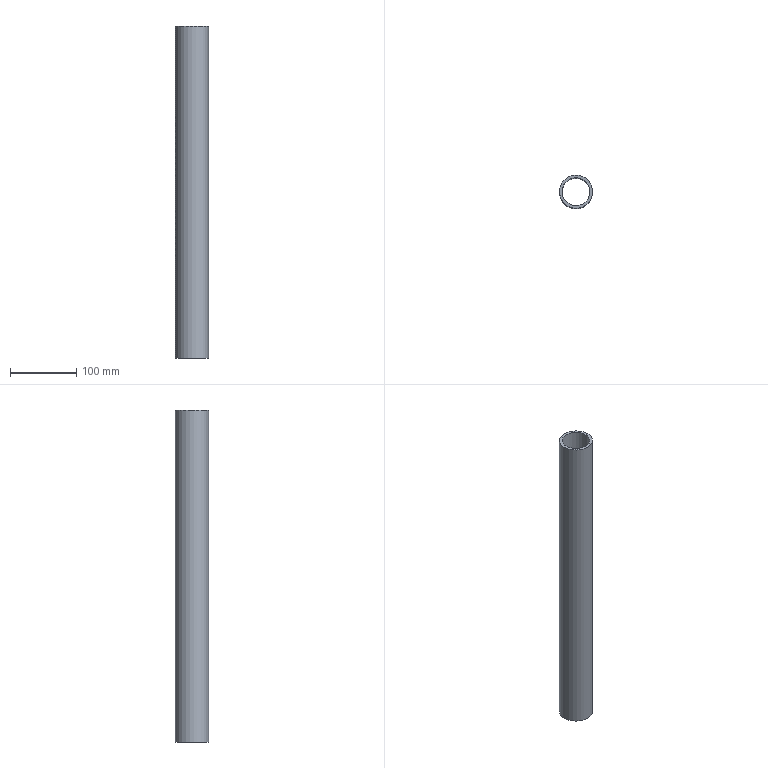Component | NX | CONN_POST_2 | 1 solid | 4 faces | box 50 x 50 x 500 mm | volume 289027 mm3 | cylinder 2 | plane 2 | commonest cylinder face diameters 50 x1 42 x1
STEP:
#1=CARTESIAN_POINT('',(0.,0.,0.));
#2=DIRECTION('',(0.,0.,1.));
#3=DIRECTION('',(1.,0.,0.));
#4=AXIS2_PLACEMENT_3D('',#1,#2,#3);
#5=CARTESIAN_POINT('',(-1330.929,336.326,-611.8));
#6=VERTEX_POINT('',#5);
#7=CARTESIAN_POINT('',(-1310.,350.,-611.8));
#8=DIRECTION('',(0.,0.,1.));
#9=DIRECTION('',(-0.8372,-0.5469,0.));
#10=AXIS2_PLACEMENT_3D('',#7,#8,#9);
#11=CIRCLE('',#10,25.);
#12=CARTESIAN_POINT('',(-1310.,350.,-611.8));
#13=DIRECTION('',(0.,0.,1.));
#14=DIRECTION('',(0.8372,0.5469,0.));
#15=AXIS2_PLACEMENT_3D('',#12,#13,#14);
#16=CYLINDRICAL_SURFACE('',#15,25.);
#17=CARTESIAN_POINT('',(3.142,0.));
#18=DIRECTION('',(1.,0.));
#19=VECTOR('',#18,1.);
#20=LINE('',#17,#19);
#21=(GEOMETRIC_REPRESENTATION_CONTEXT(2)PARAMETRIC_REPRESENTATION_CONTEXT()REPRESENTATION_CONTEXT('',''));
#22=DEFINITIONAL_REPRESENTATION('',(#20),#21);
#23=PCURVE('',#16,#22);
#24=CARTESIAN_POINT('',(-1310.,350.,-611.8));
#25=DIRECTION('',(0.,0.,1.));
#26=DIRECTION('',(0.8372,0.5469,0.));
#27=AXIS2_PLACEMENT_3D('',#24,#25,#26);
#28=PLANE('',#27);
#29=CARTESIAN_POINT('',(0.,0.));
#30=DIRECTION('',(-1.,0.));
#31=AXIS2_PLACEMENT_2D('',#29,#30);
#32=CIRCLE('',#31,25.);
#33=(GEOMETRIC_REPRESENTATION_CONTEXT(2)PARAMETRIC_REPRESENTATION_CONTEXT()REPRESENTATION_CONTEXT('',''));
#34=DEFINITIONAL_REPRESENTATION('',(#32),#33);
#35=PCURVE('',#28,#34);
#36=SURFACE_CURVE('',#11,(#23,#35),.PCURVE_S1.);
#37=EDGE_CURVE('',#6,#6,#36,.T.);
#38=ORIENTED_EDGE('',*,*,#37,.T.);
#39=CARTESIAN_POINT('',(-1330.929,336.326,-111.8));
#40=VERTEX_POINT('',#39);
#41=CARTESIAN_POINT('',(-1330.929,336.326,-611.8));
#42=CARTESIAN_POINT('',(-1330.929,336.326,-111.8));
#43=B_SPLINE_CURVE_WITH_KNOTS('',1,(#41,#42),.UNSPECIFIED.,.F.,.F.,(2,2),(0.,500.),.PIECEWISE_BEZIER_KNOTS.);
#44=CARTESIAN_POINT('',(9.425,0.));
#45=DIRECTION('',(0.,1.));
#46=VECTOR('',#45,1.);
#47=LINE('',#44,#46);
#48=(GEOMETRIC_REPRESENTATION_CONTEXT(2)PARAMETRIC_REPRESENTATION_CONTEXT()REPRESENTATION_CONTEXT('',''));
#49=DEFINITIONAL_REPRESENTATION('',(#47),#48);
#50=PCURVE('',#16,#49);
#51=CARTESIAN_POINT('',(3.142,0.));
#52=DIRECTION('',(0.,1.));
#53=VECTOR('',#52,1.);
#54=LINE('',#51,#53);
#55=(GEOMETRIC_REPRESENTATION_CONTEXT(2)PARAMETRIC_REPRESENTATION_CONTEXT()REPRESENTATION_CONTEXT('',''));
#56=DEFINITIONAL_REPRESENTATION('',(#54),#55);
#57=PCURVE('',#16,#56);
#58=SEAM_CURVE('',#43,(#50,#57),.PCURVE_S1.);
#59=EDGE_CURVE('',#6,#40,#58,.T.);
#60=ORIENTED_EDGE('',*,*,#59,.T.);
#61=CARTESIAN_POINT('',(-1310.,350.,-111.8));
#62=DIRECTION('',(0.,0.,1.));
#63=DIRECTION('',(-0.8372,-0.5469,0.));
#64=AXIS2_PLACEMENT_3D('',#61,#62,#63);
#65=CIRCLE('',#64,25.);
#66=CARTESIAN_POINT('',(3.142,500.));
#67=DIRECTION('',(1.,0.));
#68=VECTOR('',#67,1.);
#69=LINE('',#66,#68);
#70=(GEOMETRIC_REPRESENTATION_CONTEXT(2)PARAMETRIC_REPRESENTATION_CONTEXT()REPRESENTATION_CONTEXT('',''));
#71=DEFINITIONAL_REPRESENTATION('',(#69),#70);
#72=PCURVE('',#16,#71);
#73=CARTESIAN_POINT('',(-1310.,350.,-111.8));
#74=DIRECTION('',(0.,0.,1.));
#75=DIRECTION('',(0.8372,0.5469,0.));
#76=AXIS2_PLACEMENT_3D('',#73,#74,#75);
#77=PLANE('',#76);
#78=CARTESIAN_POINT('',(0.,0.));
#79=DIRECTION('',(-1.,0.));
#80=AXIS2_PLACEMENT_2D('',#78,#79);
#81=CIRCLE('',#80,25.);
#82=(GEOMETRIC_REPRESENTATION_CONTEXT(2)PARAMETRIC_REPRESENTATION_CONTEXT()REPRESENTATION_CONTEXT('',''));
#83=DEFINITIONAL_REPRESENTATION('',(#81),#82);
#84=PCURVE('',#77,#83);
#85=SURFACE_CURVE('',#65,(#72,#84),.PCURVE_S1.);
#86=EDGE_CURVE('',#40,#40,#85,.T.);
#87=ORIENTED_EDGE('',*,*,#86,.F.);
#88=ORIENTED_EDGE('',*,*,#59,.F.);
#89=EDGE_LOOP('',(#38,#60,#87,#88));
#90=FACE_BOUND('',#89,.T.);
#91=ADVANCED_FACE('',(#90),#16,.T.);
#92=CARTESIAN_POINT('',(-1327.581,338.514,-611.8));
#93=VERTEX_POINT('',#92);
#94=CARTESIAN_POINT('',(-1310.,350.,-611.8));
#95=DIRECTION('',(0.,0.,1.));
#96=DIRECTION('',(-0.8372,-0.5469,0.));
#97=AXIS2_PLACEMENT_3D('',#94,#95,#96);
#98=CIRCLE('',#97,21.);
#99=CARTESIAN_POINT('',(-1310.,350.,-611.8));
#100=DIRECTION('',(0.,0.,1.));
#101=DIRECTION('',(0.8372,0.5469,0.));
#102=AXIS2_PLACEMENT_3D('',#99,#100,#101);
#103=CYLINDRICAL_SURFACE('',#102,21.);
#104=CARTESIAN_POINT('',(3.142,0.));
#105=DIRECTION('',(1.,0.));
#106=VECTOR('',#105,1.);
#107=LINE('',#104,#106);
#108=(GEOMETRIC_REPRESENTATION_CONTEXT(2)PARAMETRIC_REPRESENTATION_CONTEXT()REPRESENTATION_CONTEXT('',''));
#109=DEFINITIONAL_REPRESENTATION('',(#107),#108);
#110=PCURVE('',#103,#109);
#111=CARTESIAN_POINT('',(0.,0.));
#112=DIRECTION('',(-1.,0.));
#113=AXIS2_PLACEMENT_2D('',#111,#112);
#114=CIRCLE('',#113,21.);
#115=(GEOMETRIC_REPRESENTATION_CONTEXT(2)PARAMETRIC_REPRESENTATION_CONTEXT()REPRESENTATION_CONTEXT('',''));
#116=DEFINITIONAL_REPRESENTATION('',(#114),#115);
#117=PCURVE('',#28,#116);
#118=SURFACE_CURVE('',#98,(#110,#117),.PCURVE_S1.);
#119=EDGE_CURVE('',#93,#93,#118,.T.);
#120=ORIENTED_EDGE('',*,*,#119,.T.);
#121=CARTESIAN_POINT('',(-1327.581,338.514,-111.8));
#122=VERTEX_POINT('',#121);
#123=CARTESIAN_POINT('',(-1327.581,338.514,-611.8));
#124=CARTESIAN_POINT('',(-1327.581,338.514,-111.8));
#125=B_SPLINE_CURVE_WITH_KNOTS('',1,(#123,#124),.UNSPECIFIED.,.F.,.F.,(2,2),(0.,500.),.PIECEWISE_BEZIER_KNOTS.);
#126=CARTESIAN_POINT('',(9.425,0.));
#127=DIRECTION('',(0.,1.));
#128=VECTOR('',#127,1.);
#129=LINE('',#126,#128);
#130=(GEOMETRIC_REPRESENTATION_CONTEXT(2)PARAMETRIC_REPRESENTATION_CONTEXT()REPRESENTATION_CONTEXT('',''));
#131=DEFINITIONAL_REPRESENTATION('',(#129),#130);
#132=PCURVE('',#103,#131);
#133=CARTESIAN_POINT('',(3.142,0.));
#134=DIRECTION('',(0.,1.));
#135=VECTOR('',#134,1.);
#136=LINE('',#133,#135);
#137=(GEOMETRIC_REPRESENTATION_CONTEXT(2)PARAMETRIC_REPRESENTATION_CONTEXT()REPRESENTATION_CONTEXT('',''));
#138=DEFINITIONAL_REPRESENTATION('',(#136),#137);
#139=PCURVE('',#103,#138);
#140=SEAM_CURVE('',#125,(#132,#139),.PCURVE_S1.);
#141=EDGE_CURVE('',#93,#122,#140,.T.);
#142=ORIENTED_EDGE('',*,*,#141,.T.);
#143=CARTESIAN_POINT('',(-1310.,350.,-111.8));
#144=DIRECTION('',(0.,0.,1.));
#145=DIRECTION('',(-0.8372,-0.5469,0.));
#146=AXIS2_PLACEMENT_3D('',#143,#144,#145);
#147=CIRCLE('',#146,21.);
#148=CARTESIAN_POINT('',(3.142,500.));
#149=DIRECTION('',(1.,0.));
#150=VECTOR('',#149,1.);
#151=LINE('',#148,#150);
#152=(GEOMETRIC_REPRESENTATION_CONTEXT(2)PARAMETRIC_REPRESENTATION_CONTEXT()REPRESENTATION_CONTEXT('',''));
#153=DEFINITIONAL_REPRESENTATION('',(#151),#152);
#154=PCURVE('',#103,#153);
#155=CARTESIAN_POINT('',(0.,0.));
#156=DIRECTION('',(-1.,0.));
#157=AXIS2_PLACEMENT_2D('',#155,#156);
#158=CIRCLE('',#157,21.);
#159=(GEOMETRIC_REPRESENTATION_CONTEXT(2)PARAMETRIC_REPRESENTATION_CONTEXT()REPRESENTATION_CONTEXT('',''));
#160=DEFINITIONAL_REPRESENTATION('',(#158),#159);
#161=PCURVE('',#77,#160);
#162=SURFACE_CURVE('',#147,(#154,#161),.PCURVE_S1.);
#163=EDGE_CURVE('',#122,#122,#162,.T.);
#164=ORIENTED_EDGE('',*,*,#163,.F.);
#165=ORIENTED_EDGE('',*,*,#141,.F.);
#166=EDGE_LOOP('',(#120,#142,#164,#165));
#167=FACE_BOUND('',#166,.F.);
#168=ADVANCED_FACE('',(#167),#103,.F.);
#169=ORIENTED_EDGE('',*,*,#37,.F.);
#170=EDGE_LOOP('',(#169));
#171=FACE_BOUND('',#170,.T.);
#172=ORIENTED_EDGE('',*,*,#119,.T.);
#173=EDGE_LOOP('',(#172));
#174=FACE_BOUND('',#173,.T.);
#175=ADVANCED_FACE('',(#171,#174),#28,.F.);
#176=ORIENTED_EDGE('',*,*,#86,.T.);
#177=EDGE_LOOP('',(#176));
#178=FACE_BOUND('',#177,.T.);
#179=ORIENTED_EDGE('',*,*,#163,.F.);
#180=EDGE_LOOP('',(#179));
#181=FACE_BOUND('',#180,.T.);
#182=ADVANCED_FACE('',(#178,#181),#77,.T.);
#183=CLOSED_SHELL('',(#91,#168,#175,#182));
#184=MANIFOLD_SOLID_BREP('',#183);
#185=(LENGTH_UNIT()NAMED_UNIT(*)SI_UNIT(.MILLI.,.METRE.));
#186=UNCERTAINTY_MEASURE_WITH_UNIT(LENGTH_MEASURE(0.00001),#185,'','');
#187=(NAMED_UNIT(*)PLANE_ANGLE_UNIT()SI_UNIT($,.RADIAN.));
#188=(NAMED_UNIT(*)SI_UNIT($,.STERADIAN.)SOLID_ANGLE_UNIT());
#189=(GEOMETRIC_REPRESENTATION_CONTEXT(3)GLOBAL_UNCERTAINTY_ASSIGNED_CONTEXT((#186))GLOBAL_UNIT_ASSIGNED_CONTEXT((#185,#187,#188))REPRESENTATION_CONTEXT('',''));
#190=ADVANCED_BREP_SHAPE_REPRESENTATION('',(#4,#184),#189);